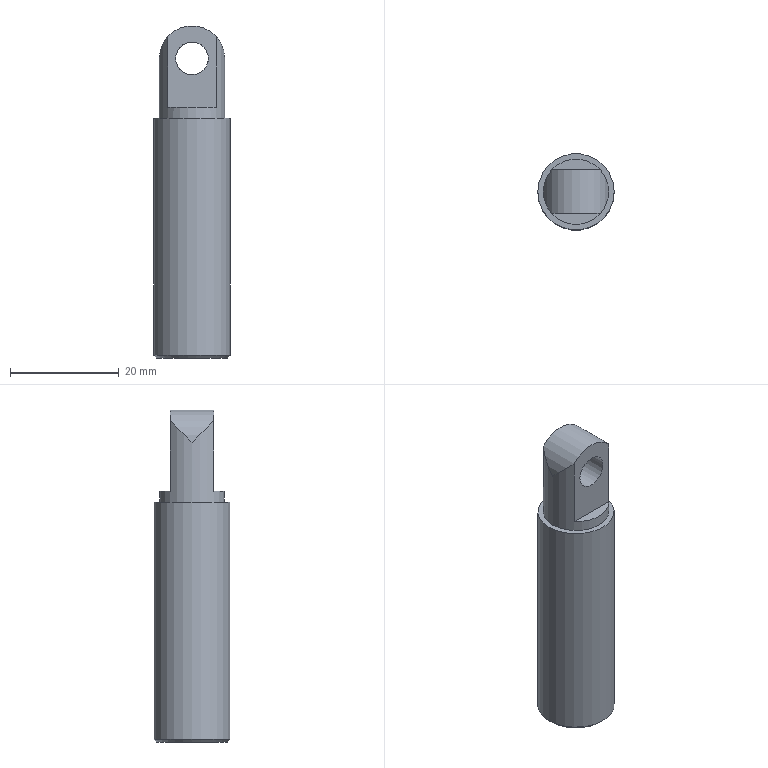Component | NX | 5 | 1 solid | 18 faces | volume 7635 mm3 | plane 8 | cylinder 6 | spline 3 | cone 1 | commonest cylinder face diameters 12 x2 6 x2 5 x1 14 x1